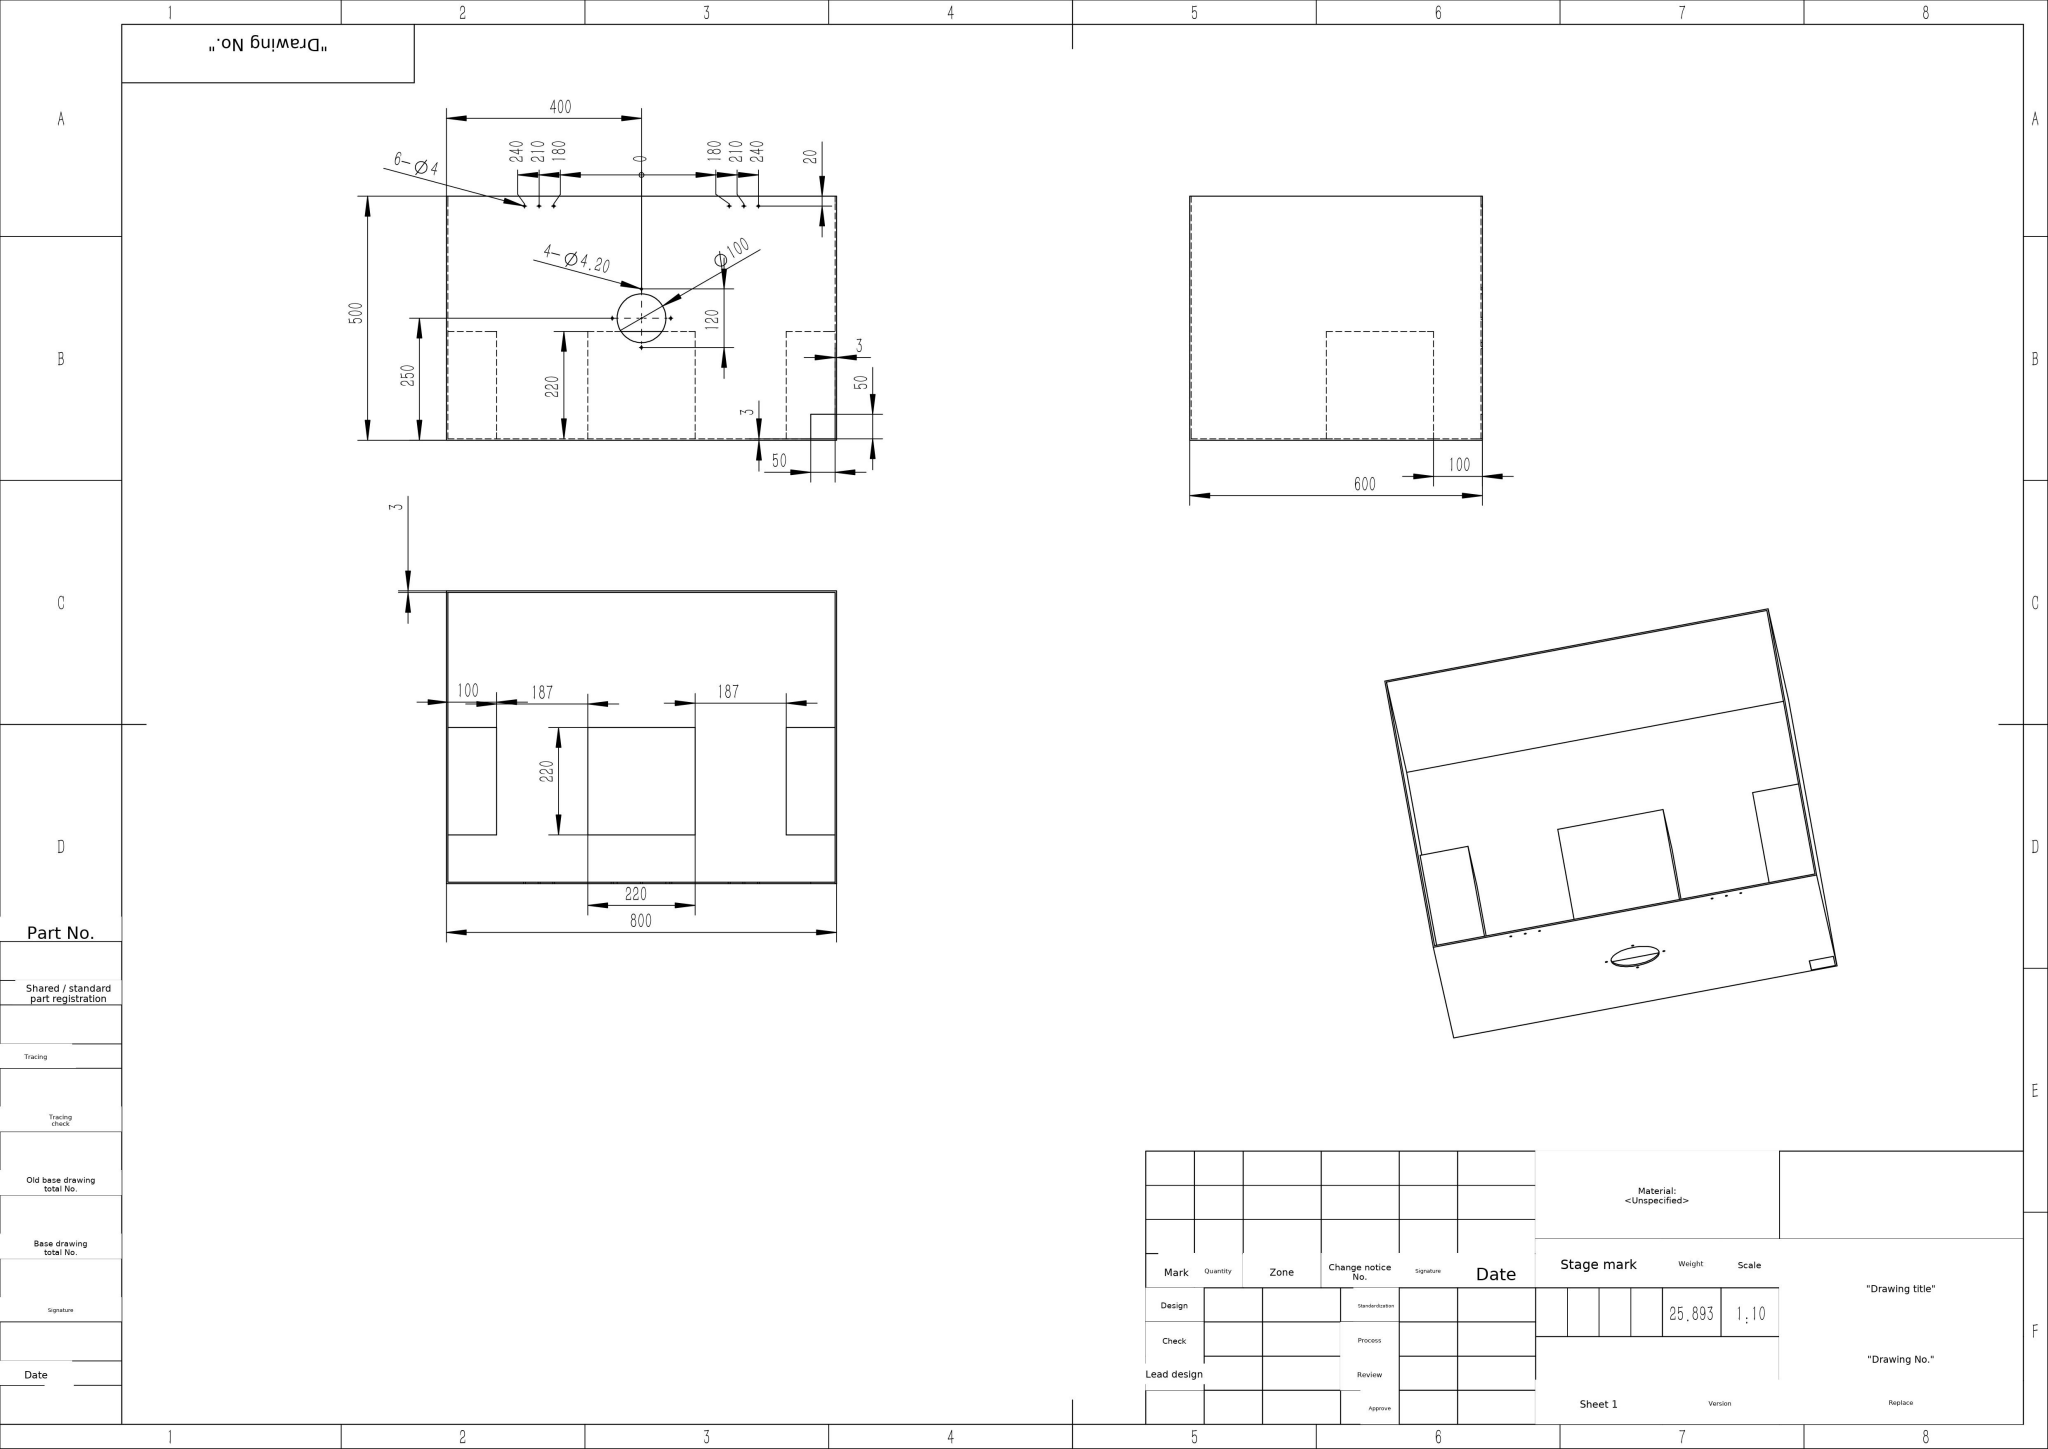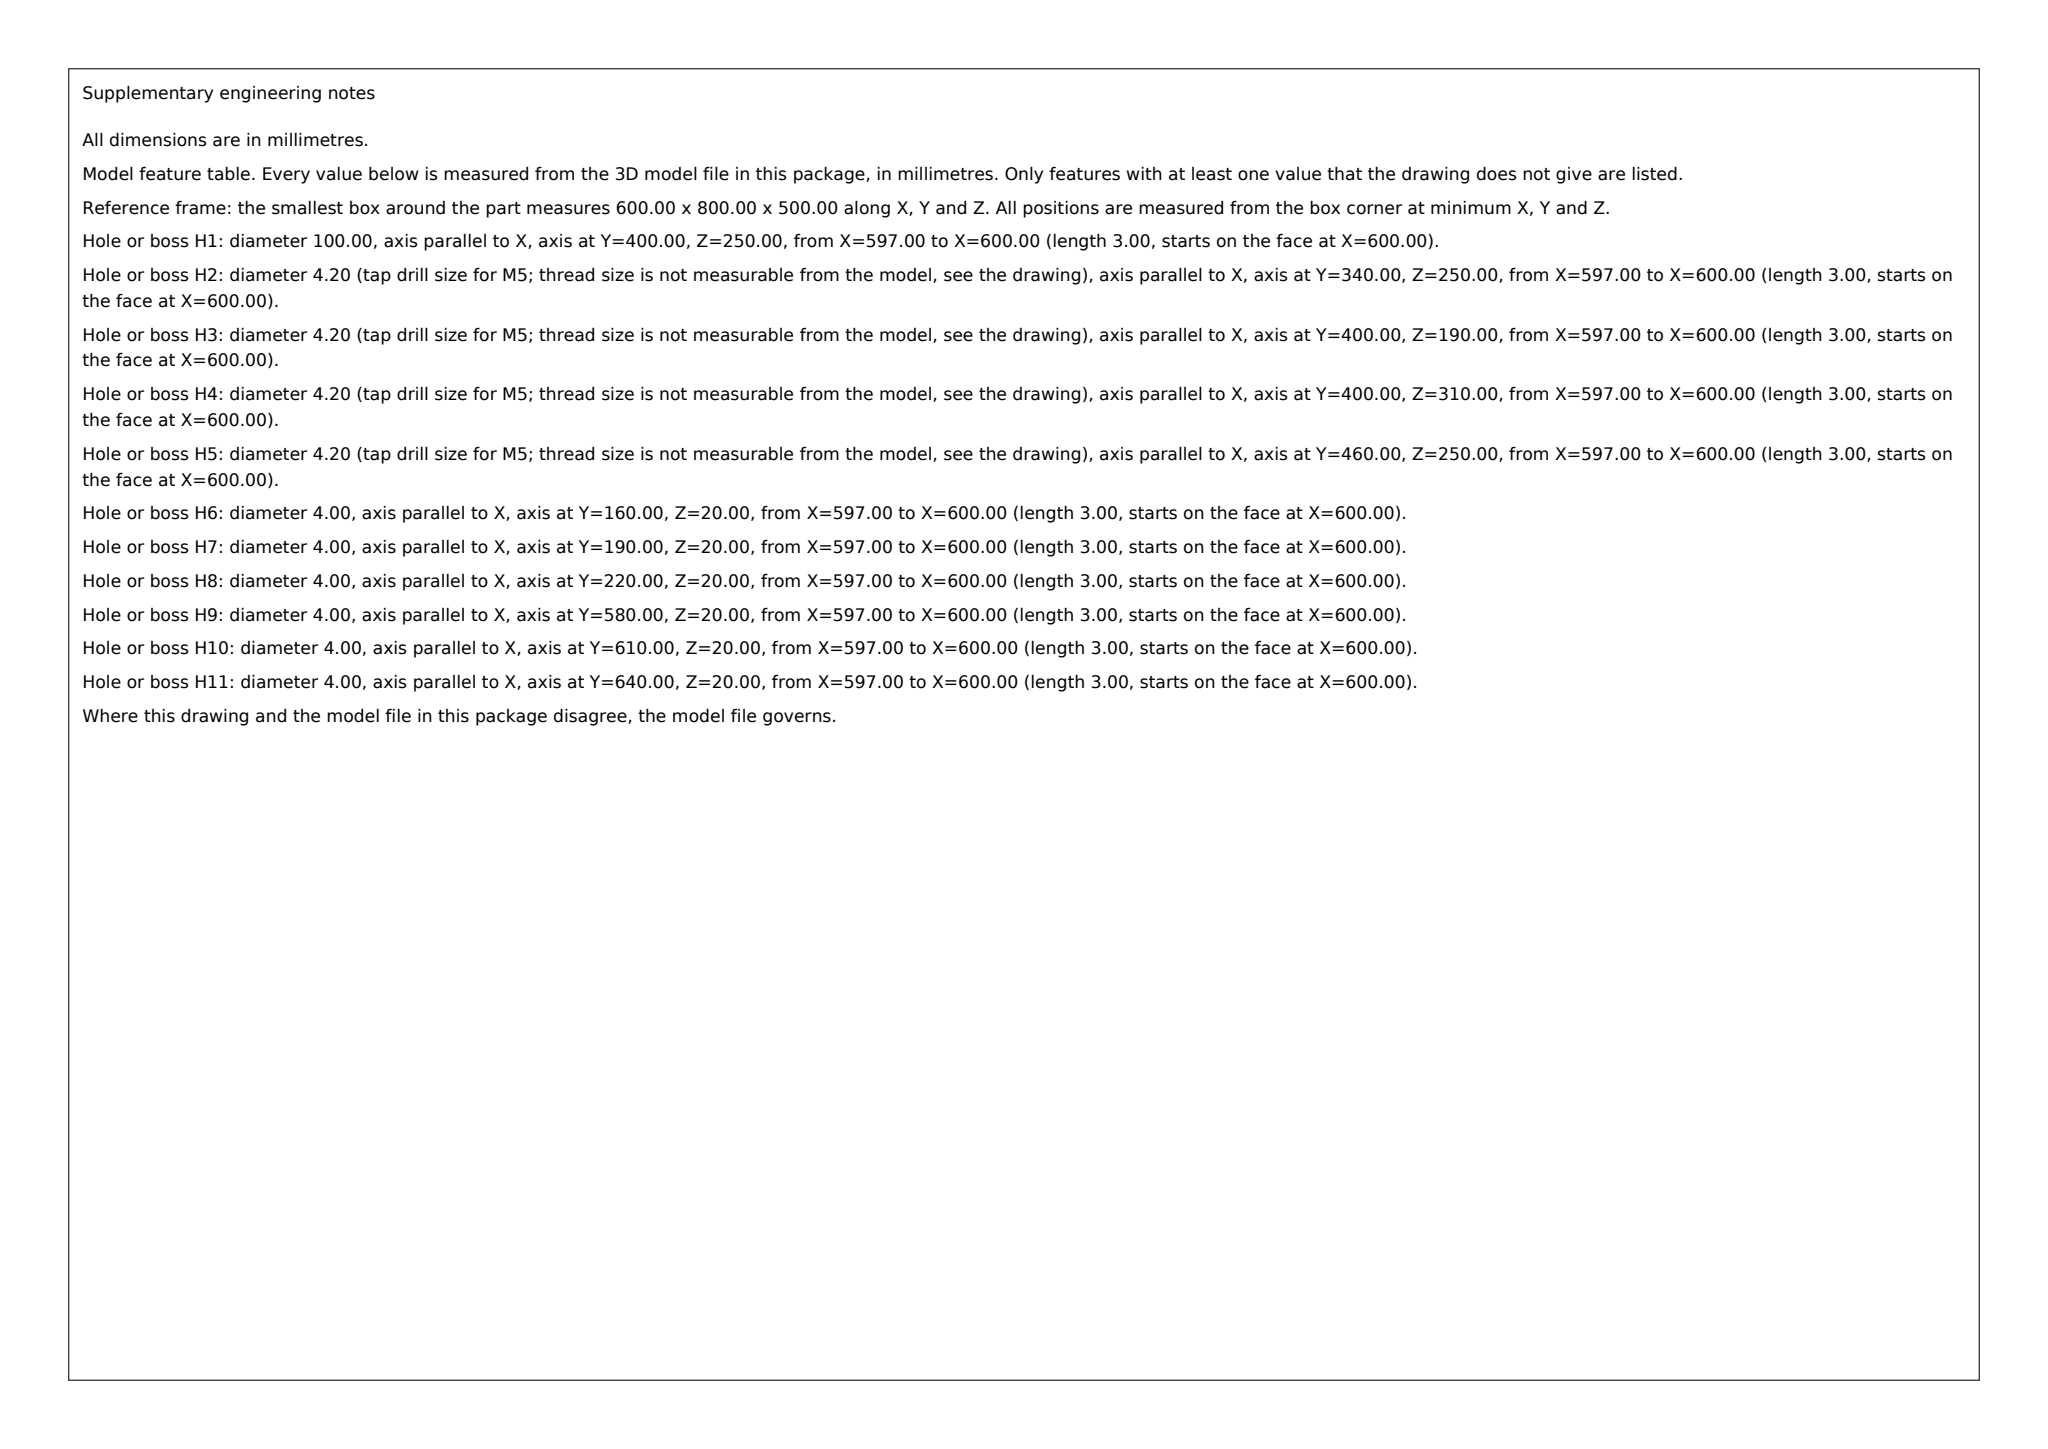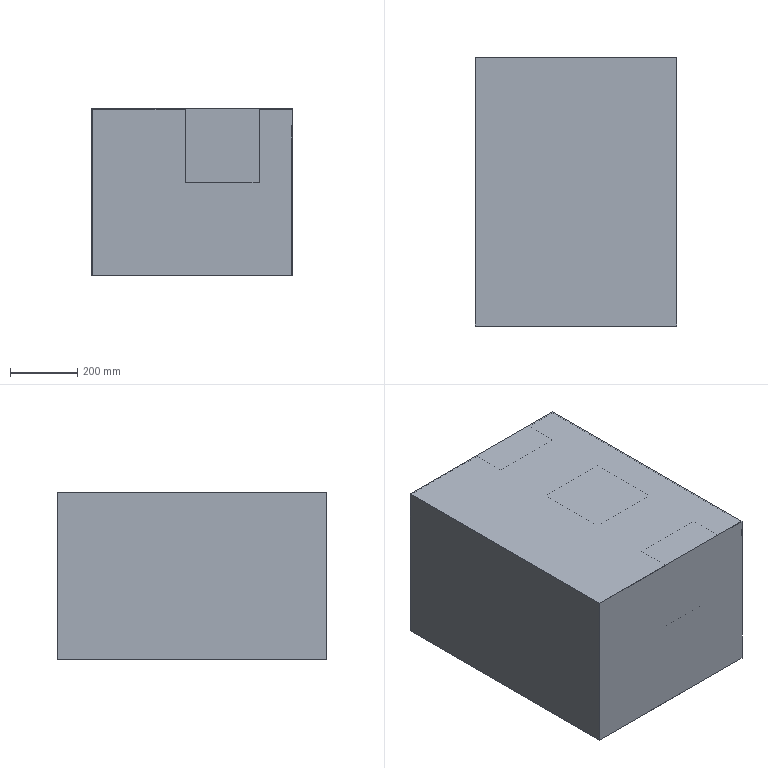Part | SolidWorks | mm | 1 solid | 48 faces | box 600 x 800 x 500 mm | volume 25893454 mm3 | plane 26 | cylinder 22 | commonest cylinder face diameters 4 x12 4.2 x8 100 x2
build123d program:
from build123d import *

# Parameters (mm, degrees)
SKETCH1_W                     = 600
SKETCH1_H                     = 500
BOSS_EXTRUDE1_DEPTH           = 800
SHELL1_T                      = -3
SKETCH2_W                     = 220
SKETCH2_H                     = 220
SKETCH2_H_2                   = 100
BOSS_EXTRUDE2_DEPTH           = 220
SKETCH3_R                     = 50
CUT_EXTRUDE1_DEPTH            = 10
SKETCH4_R                     = 2.1
CUT_EXTRUDE3_DEPTH            = 10
CIRPATTERN1_COUNT             = 4
SKETCH6_W                     = 50
SKETCH6_H                     = 50
CUT_EXTRUDE4_DEPTH            = 10
SIZE_MM_DOWEL_PIN_HOLE1_D     = 4
SIZE_MM_DOWEL_PIN_HOLE1_DEPTH = 5.16
SIZE_MM_DOWEL_PIN_HOLE1_TIP   = 1.202


with BuildPart() as part:
    # Sketch1 → Boss-Extrude1 (new body)
    with BuildSketch(Plane(origin=(0, 0, 0), x_dir=(1, 0, 0), z_dir=(0, 1, 0))):
        Rectangle(SKETCH1_W, SKETCH1_H)
    extrude(amount=BOSS_EXTRUDE1_DEPTH)

    # Shell1
    shell1_openings = [part.faces().sort_by_distance(p)[0] for p in [
        (0, 400, -250),
    ]]
    offset(amount=SHELL1_T, openings=shell1_openings, kind=Kind.INTERSECTION)

    # Sketch2 → Boss-Extrude2 (add)
    with BuildSketch(Plane(origin=(0, 0, 247), x_dir=(-1, 0, 0), z_dir=(0, 0, -1))):
        with Locations((-90, 400)):
            Rectangle(SKETCH2_W, SKETCH2_H)
        with Locations((-90, 53)):
            Rectangle(SKETCH2_W, SKETCH2_H_2)
        with Locations((-90, 747)):
            Rectangle(SKETCH2_W, SKETCH2_H_2)
    extrude(amount=BOSS_EXTRUDE2_DEPTH)

    # Sketch3 → Cut-Extrude1 (cut)
    with BuildSketch(Plane.ZY.offset(-300)):
        with Locations((0, 400)):
            Circle(SKETCH3_R)
    extrude(amount=CUT_EXTRUDE1_DEPTH, mode=Mode.SUBTRACT)

    # Sketch4 → Cut-Extrude3 (cut)
    with BuildSketch(Plane.ZY.offset(-300)):
        with Locations((-60, 400)):
            Circle(SKETCH4_R)
    cut_extrude3 = extrude(amount=CUT_EXTRUDE3_DEPTH, mode=Mode.SUBTRACT)

    # CirPattern1: Cut-Extrude3 ×4 about axis
    cirpattern1_axis = Axis((0, 400, 0), (1, 0, 0))
    for i in range(1, CIRPATTERN1_COUNT):
        add(cut_extrude3.rotate(cirpattern1_axis, i * 360 / CIRPATTERN1_COUNT), mode=Mode.SUBTRACT)

    # Sketch6 → Cut-Extrude4 (cut)
    with BuildSketch(Plane.ZY.offset(-300)):
        with Locations((222, 28)):
            Rectangle(SKETCH6_W, SKETCH6_H)
    extrude(amount=CUT_EXTRUDE4_DEPTH, mode=Mode.SUBTRACT)

    # Size mm Dowel Pin Hole1
    with Locations(Plane(origin=(300, 0, 0), x_dir=(0, 0, -1), z_dir=(1, 0, 0))):
        with Locations((230, 640), (230, 610), (230, 580), (230, 220), (230, 190), (230, 160)):
            Hole(SIZE_MM_DOWEL_PIN_HOLE1_D / 2, depth=SIZE_MM_DOWEL_PIN_HOLE1_DEPTH)
            with Locations((0, 0, -(SIZE_MM_DOWEL_PIN_HOLE1_DEPTH + SIZE_MM_DOWEL_PIN_HOLE1_TIP / 2))):  # 118° drill point
                Cone(0, SIZE_MM_DOWEL_PIN_HOLE1_D / 2, SIZE_MM_DOWEL_PIN_HOLE1_TIP, mode=Mode.SUBTRACT)


solid = part.part